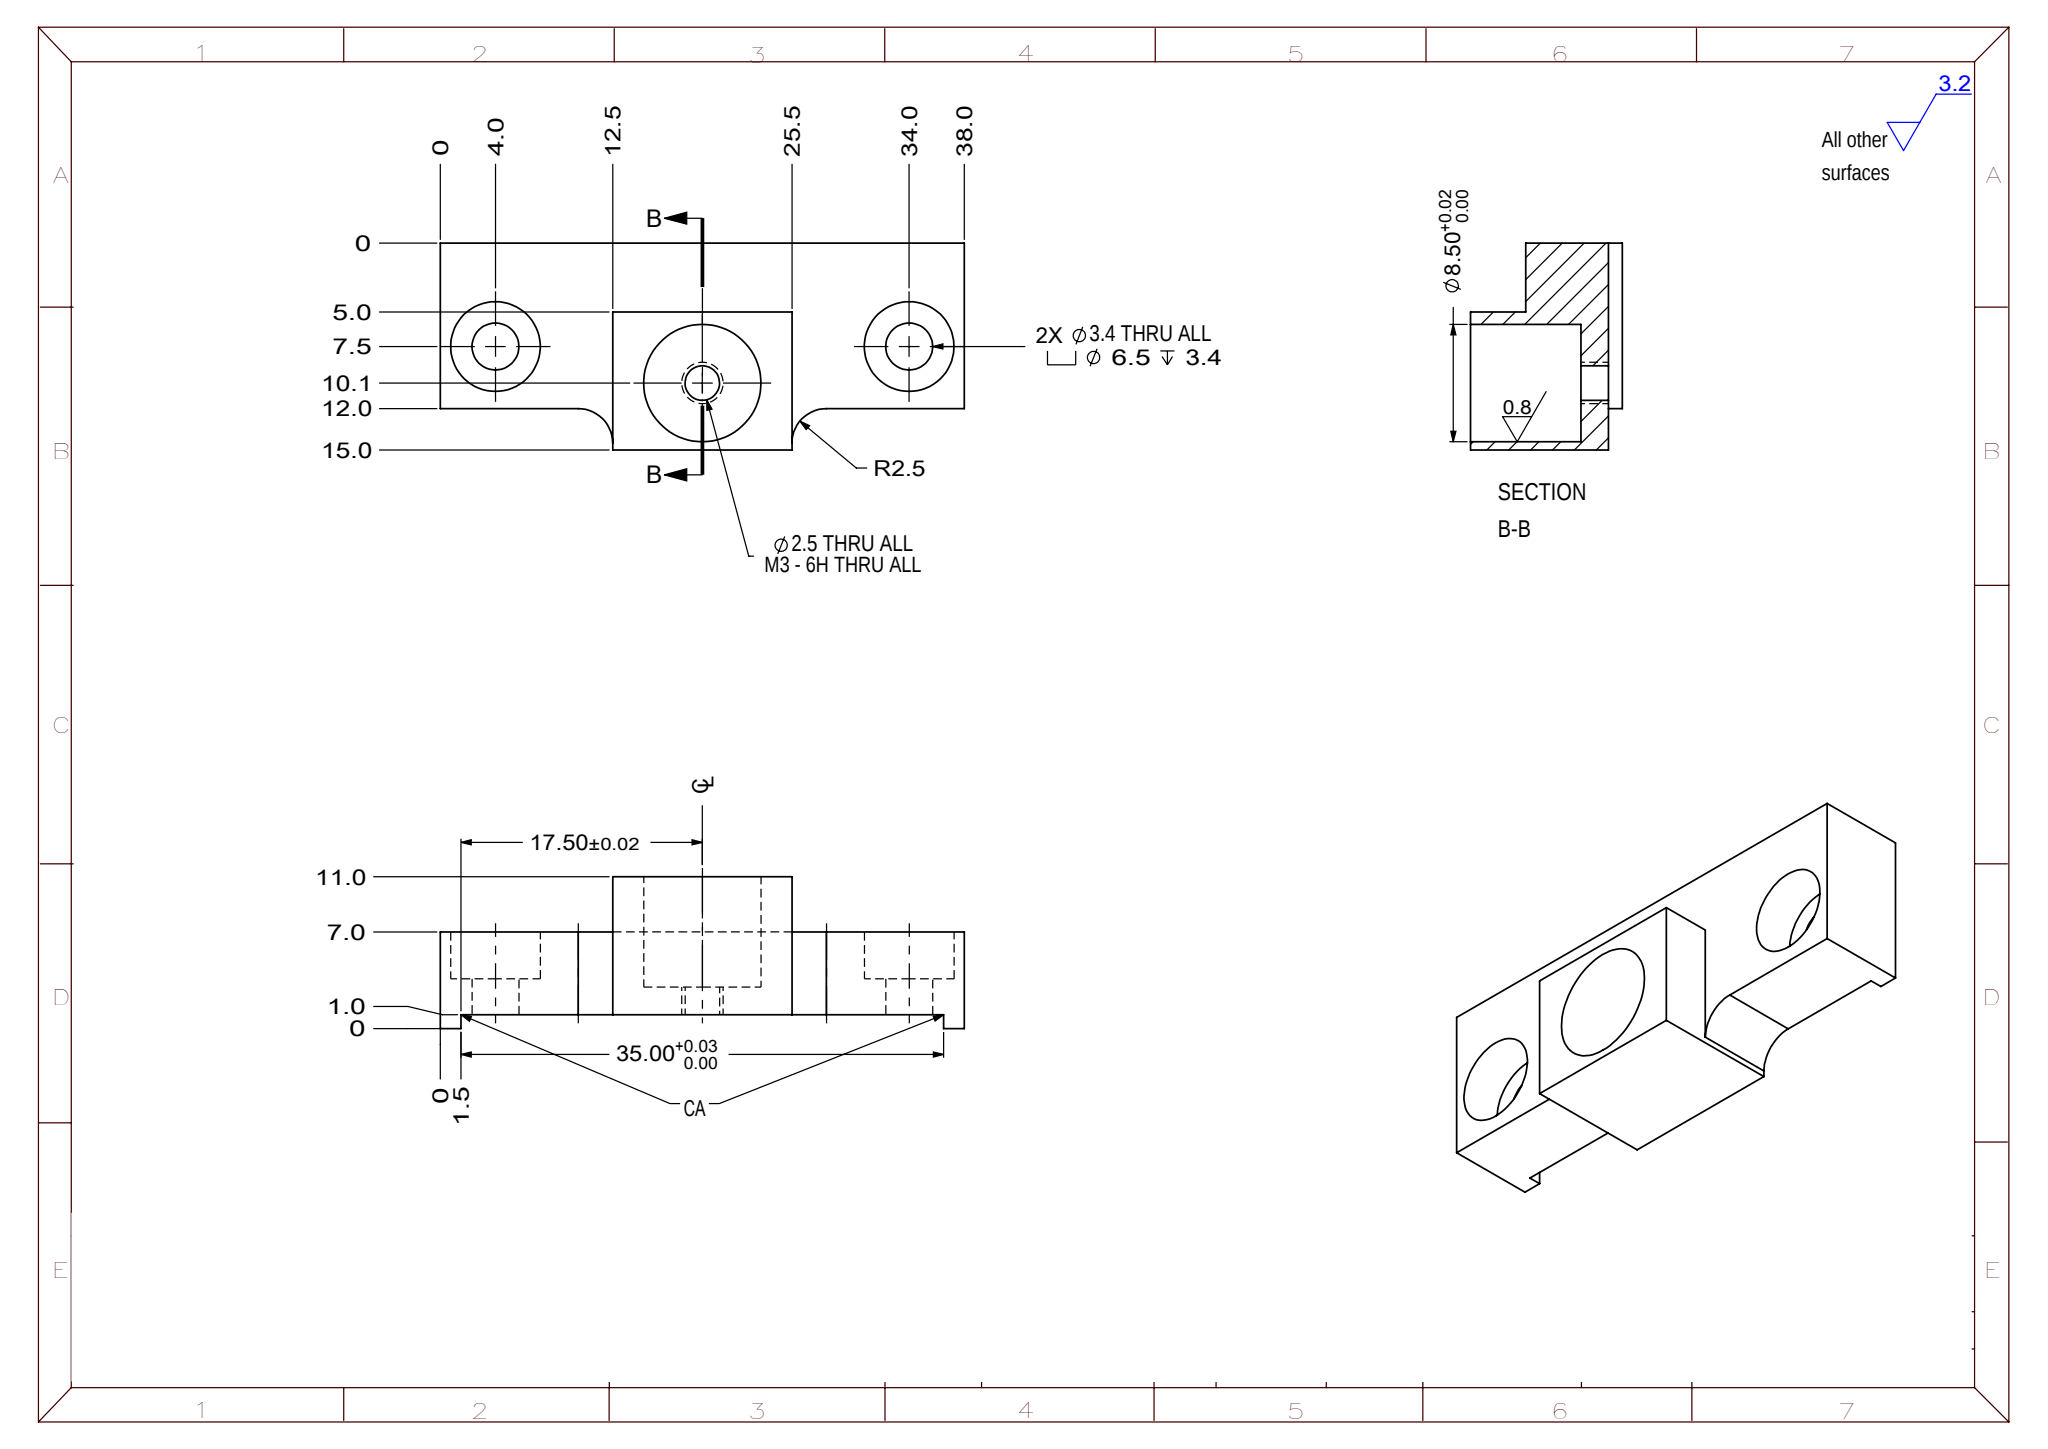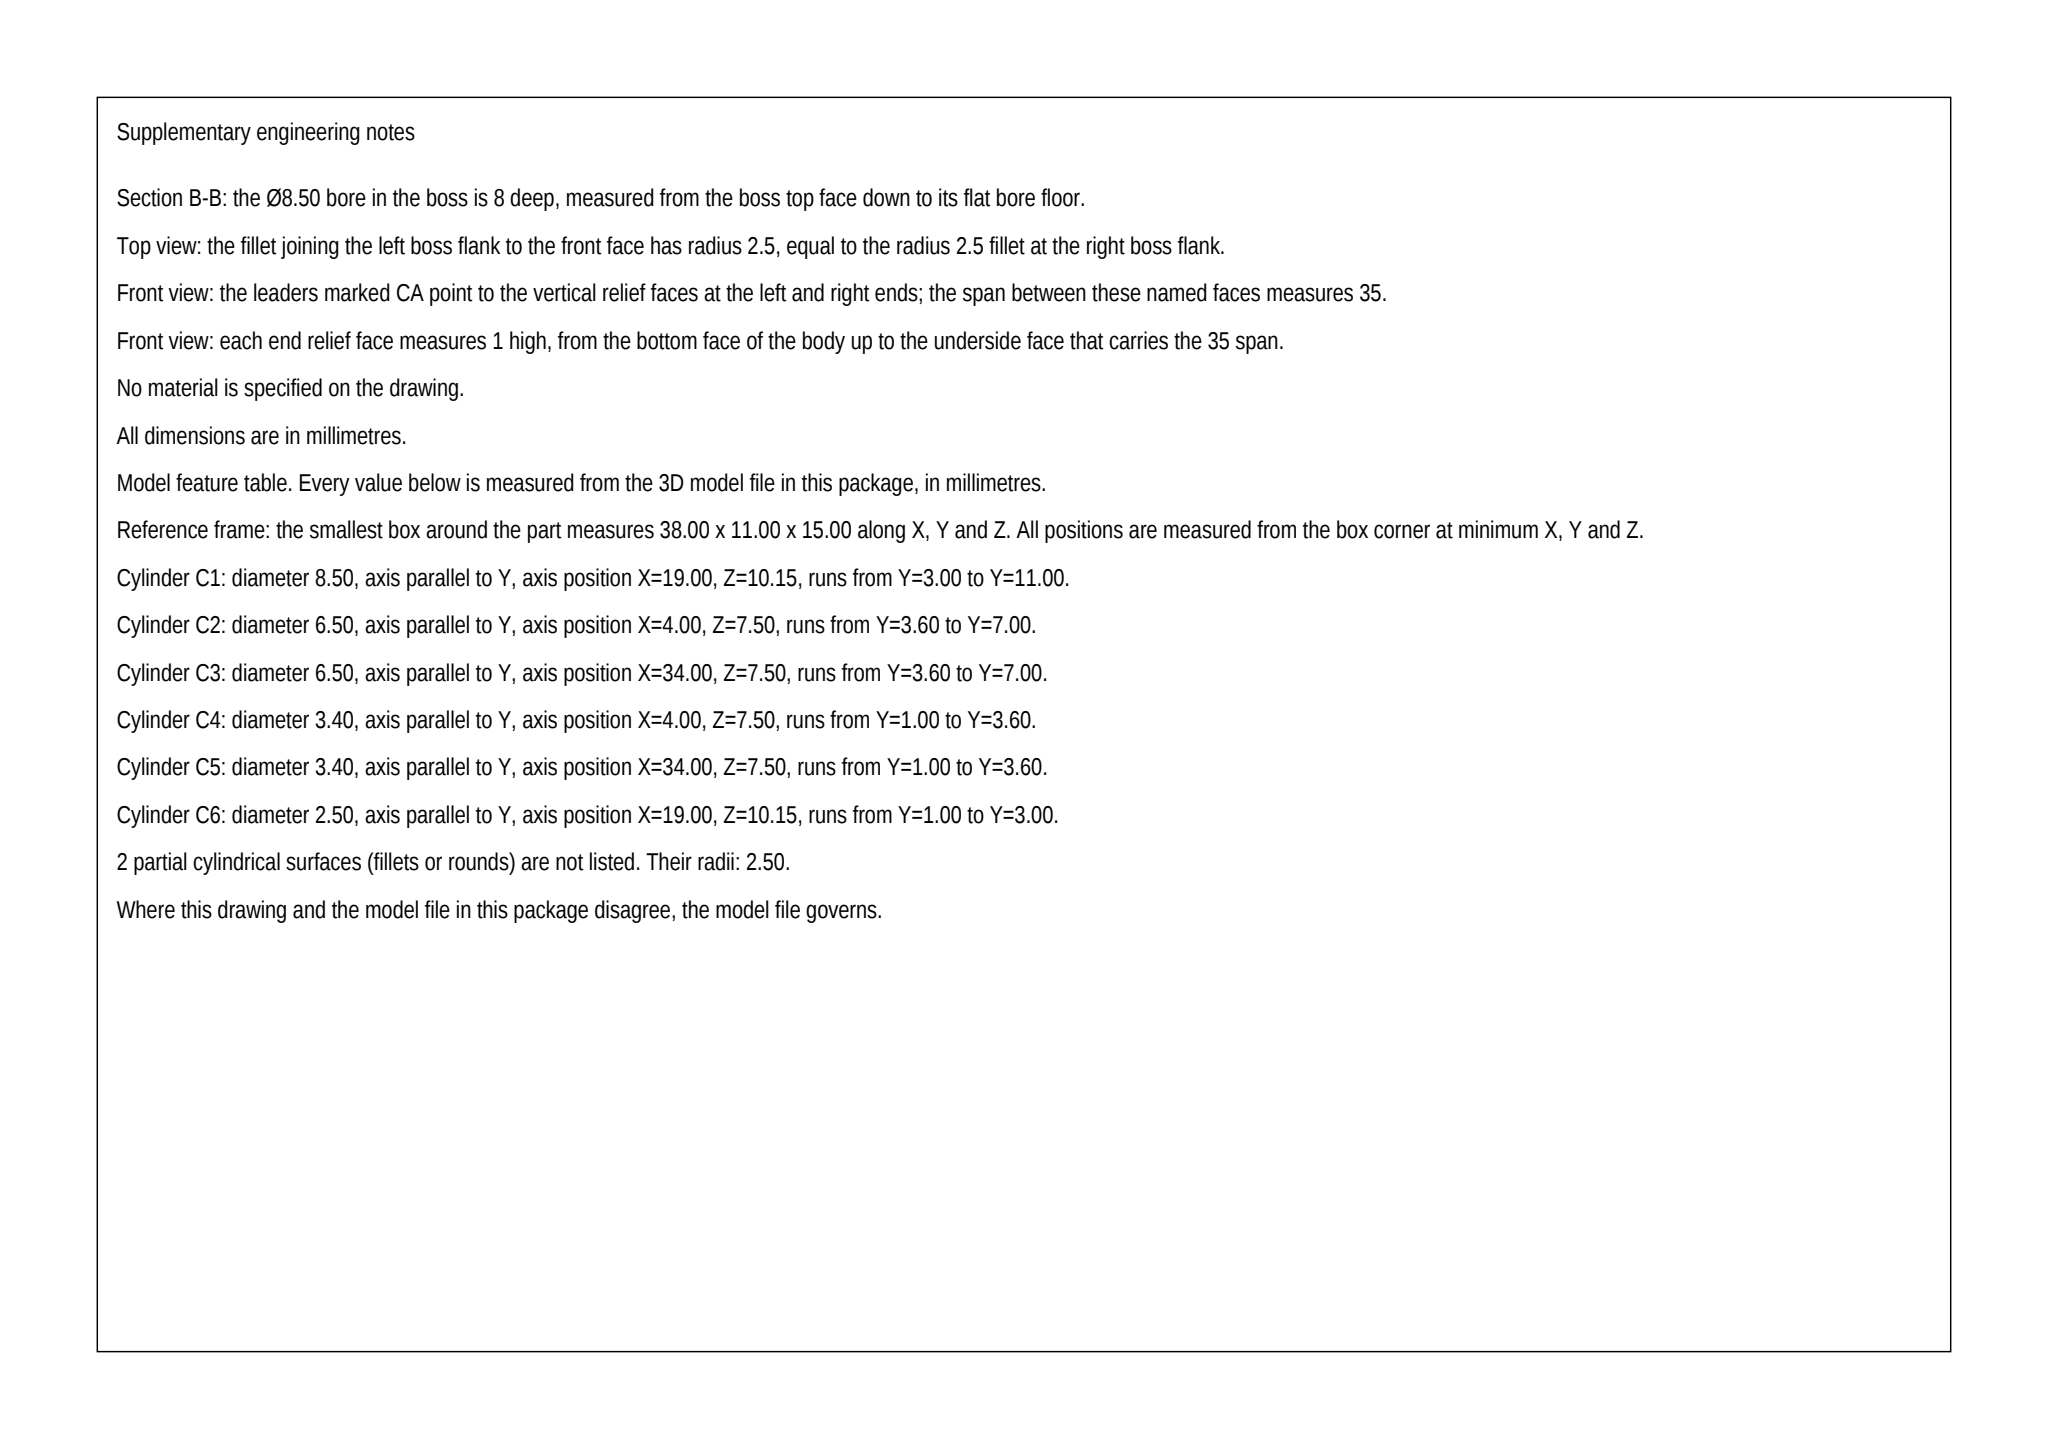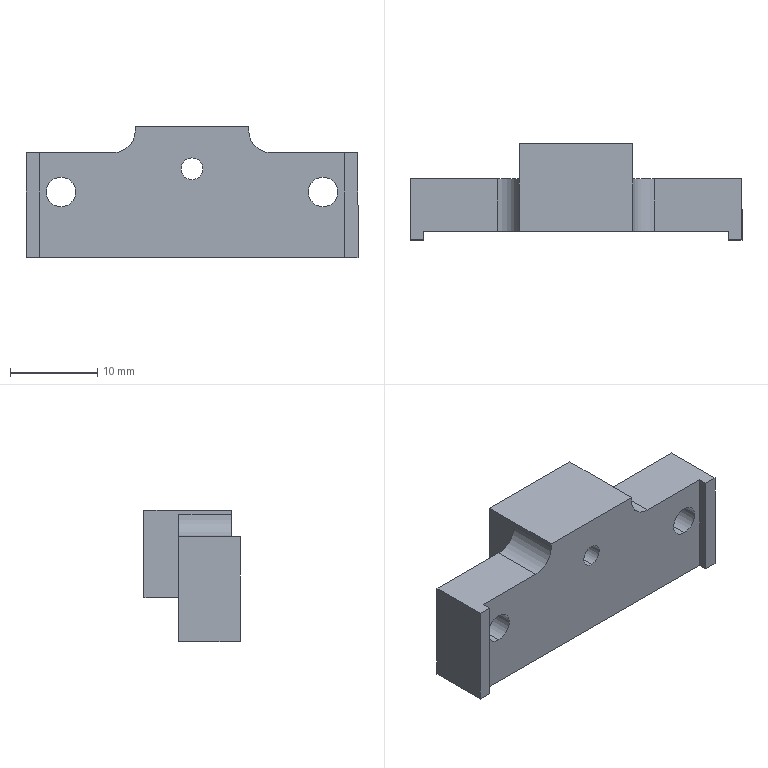Part | SolidWorks | mm | 1 solid | 33 faces | box 38 x 11 x 15 mm | volume 2805 mm3 | plane 19 | cylinder 14 | commonest cylinder face diameters 6.5 x4 3.4 x4 2.5 x2 8.5 x2 5 x2
Drawing notes:
Ø8.50 +0.02/0 bore DP 8.0 from top face (11.0 level) | from the solid: cylinder [8.5,"y",[19.0,null,10.15],8.0]; y-planes 11.0 top and 3.0 bore bottom
Ø2.5 THRU hole, located 19.0 from left end face and 10.15 from top edge (0 level); coaxial with the Ø8.50 bore. | from the solid: cylinders: [2.5, "y", [19.0, null, 10.15], 2.0] coaxial with [8.5, "y", [19.0, null, 10.15], 8.0]
Underside recess face at 3.0 above bottom face (0 level), measured parallel to the 7.0 and 11.0 levels. | from the solid: axis_planes: ["y", 3.0, 1] (with y planes 0.0, 1.0, 7.0, 11.0)
Center hole: Ø2.5 THRU, tapped M3-6H THRU; axis at X=19.0, Z=10.15 from bbox min corner | from the solid: cylinders[2.5,'y',[19.0,null,10.15],2.0,2]
Ø8.50 +0.02/0 bore coaxial with M3 hole at X=19.0, Z=10.15, DP 8.0 from top face (Y=11.0) | from the solid: cylinders[8.5,'y',[19.0,null,10.15],8.0,2]
Underside relief face at Y=3.0 above bottom face (Y=0 datum) | from the solid: axis_planes['y',3.0]
Ø2.5 THRU hole, axis at X=19.0, Z=10.15 from bbox min corner; coaxial with Ø8.50 bore (tapped M3-6H THRU) | from the solid: cylinders: [2.5,"y",[19.0,null,10.15],2.0] and [8.5,"y",[19.0,null,10.15],8.0]
Underside relief face at Y=3.0 above bottom face (Y=0 datum), parallel to 7.0 and 11.0 levels | from the solid: axis_planes: ["y",3.0,1] with ["y",0.0,2]
build123d program:
from build123d import *

# Parameters (mm, degrees)
BOSS_EXTRUDE1_DEPTH                             = 7.5
SKETCH2_W                                       = 12.5
SKETCH2_H                                       = 4
CUT_EXTRUDE1_DEPTH                              = 25.824
SKETCH3_R                                       = 4.25
CUT_EXTRUDE2_DEPTH                              = 8
SKETCH6_W                                       = 13
SKETCH6_H                                       = 5
CUT_EXTRUDE3_DEPTH                              = 4
M3_TAPPED_HOLE1_D                               = 2.5
CUT_EXTRUDE4_DEPTH                              = 22.593
M3_HEX_SOCKET_HEAD_CAP_SCREW_CBORE1_D           = 3.4
M3_HEX_SOCKET_HEAD_CAP_SCREW_CBORE1_CBORE_D     = 6.5
M3_HEX_SOCKET_HEAD_CAP_SCREW_CBORE1_CBORE_DEPTH = 3.4


with BuildPart() as part:
    # Sketch1 → Boss-Extrude1 (new, symmetric)
    with BuildSketch(Plane.XY):
        Polygon((-17.5, -5.5), (-17.5, -4.5), (17.5, -4.5), (17.5, -5.5), (19, -5.5), (19, 5.5), (-19, 5.5), (-19, -5.5), align=None)
    extrude(amount=BOSS_EXTRUDE1_DEPTH, both=True)

    # Sketch2 → Cut-Extrude1 (cut, through all)
    with BuildSketch(Plane.XY.offset(7.5)):
        with Locations((-12.75, 3.5)):
            Rectangle(SKETCH2_W, SKETCH2_H)
        with Locations((12.75, 3.5)):
            Rectangle(SKETCH2_W, SKETCH2_H)
    extrude(amount=-CUT_EXTRUDE1_DEPTH, mode=Mode.SUBTRACT)

    # Sketch3 → Cut-Extrude2 (cut)
    with BuildSketch(Plane(origin=(0, 5.5, 0), x_dir=(1, 0, 0), z_dir=(0, 1, 0))):
        with Locations(Location((0, -2.65, 0), (0, 0, 270))):
            Circle(SKETCH3_R)
    extrude(amount=-CUT_EXTRUDE2_DEPTH, mode=Mode.SUBTRACT)

    # Sketch6 → Cut-Extrude3 (cut)
    with BuildSketch(Plane(origin=(0, 5.5, 0), x_dir=(1, 0, 0), z_dir=(0, 1, 0))):
        with Locations((0, 5)):
            Rectangle(SKETCH6_W, SKETCH6_H)
    extrude(amount=-CUT_EXTRUDE3_DEPTH, mode=Mode.SUBTRACT)

    # M3 Tapped Hole1 (through all)
    with Locations(Plane(origin=(0, -2.5, 0), x_dir=(1, 0, 0), z_dir=(0, 1, 0))):
        with Locations((0, -2.65)):
            Hole(M3_TAPPED_HOLE1_D / 2)

    # Sketch7 → Cut-Extrude4 (cut, through all)
    with BuildSketch(Plane(origin=(0, 1.5, 0), x_dir=(1, 0, 0), z_dir=(0, 1, 0))):
        with BuildLine():
            Line((-19, -7.5), (-6.5, -7.5))
            Line((-6.5, -7.5), (-6.5, -7))
            ThreePointArc((-6.5, -7), (-7.232, -5.232), (-9, -4.5))
            Line((-9, -4.5), (-19, -4.5))
            Line((-19, -4.5), (-19, -7.5))
        make_face()
        with BuildLine():
            Line((6.5, -7.5), (6.5, -7))
            ThreePointArc((6.5, -7), (7.232, -5.232), (9, -4.5))
            Line((9, -4.5), (19, -4.5))
            Line((19, -4.5), (19, -7.5))
            Line((19, -7.5), (6.5, -7.5))
        make_face()
    extrude(amount=-CUT_EXTRUDE4_DEPTH, mode=Mode.SUBTRACT)

    # M3 Hex Socket Head Cap Screw CBORE1 (through all)
    with Locations(Plane(origin=(0, 1.5, 0), x_dir=(1, 0, 0), z_dir=(0, 1, 0))):
        with Locations((-15, 0), (15, 0)):
            CounterBoreHole(M3_HEX_SOCKET_HEAD_CAP_SCREW_CBORE1_D / 2, M3_HEX_SOCKET_HEAD_CAP_SCREW_CBORE1_CBORE_D / 2, M3_HEX_SOCKET_HEAD_CAP_SCREW_CBORE1_CBORE_DEPTH)


solid = part.part